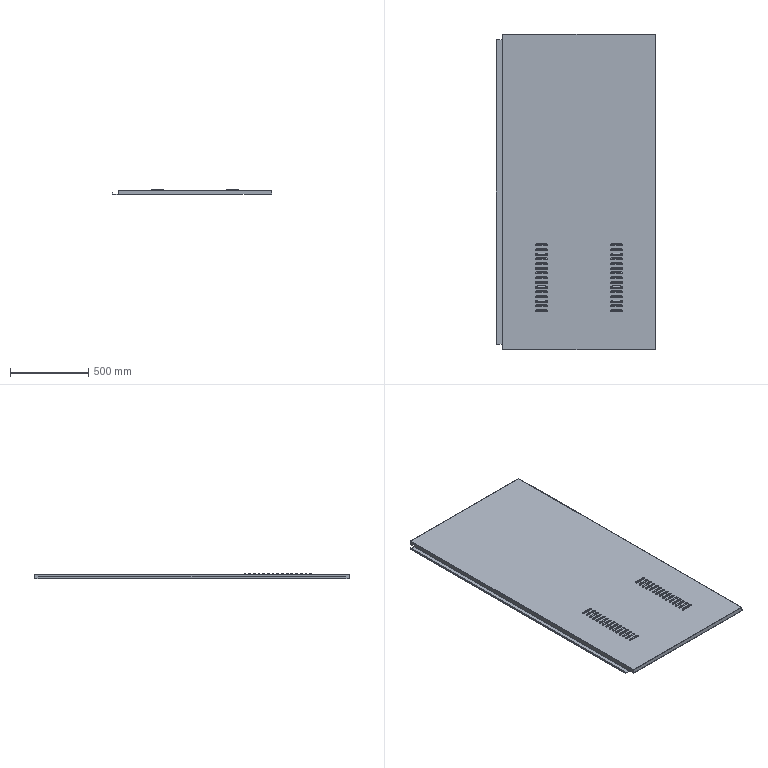Component | SolidWorks | FrontDoorPanel2-1 | 1 solid | 858 faces | volume 3390475 mm3 | cylinder 384 | torus 240 | plane 234 | commonest cylinder face diameters 8 x180 5 x90 11 x90 3.4 x12 0.4 x12